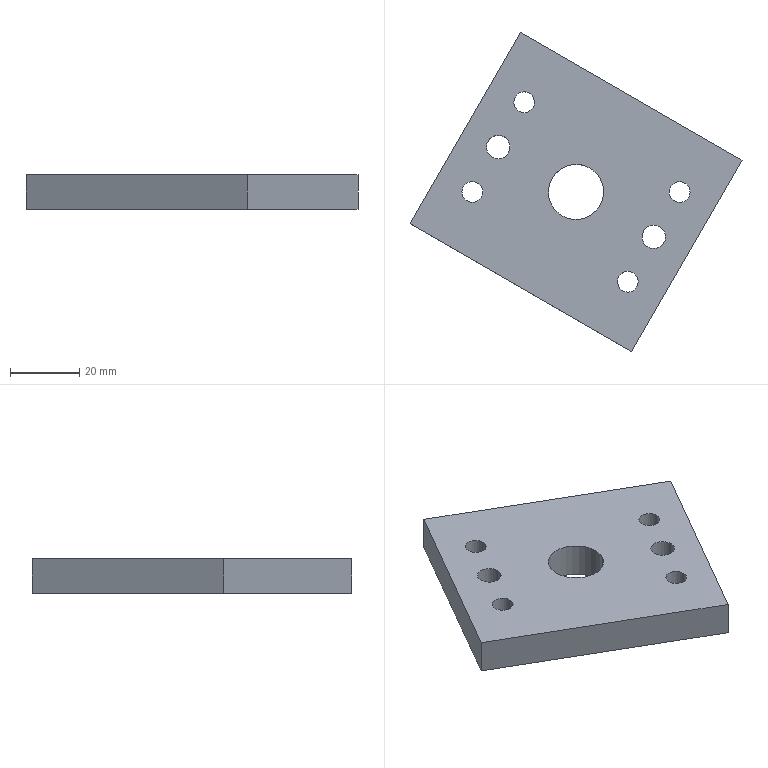Component | SolidWorks | KLHFH001LocatingPlate-1 | 1 solid | 20 faces | box 96.09 x 92.43 x 10 mm | volume 43492 mm3 | cylinder 14 | plane 6 | commonest cylinder face diameters 6 x8 6.8 x4 16 x2 | material AISI Type A2 Tool Steel
build123d program:
from build123d import *

# Parameters (mm, degrees)
SKETCH1_W                 = 74
SKETCH1_H                 = 64
BOSS_EXTRUDE1_DEPTH       = 5
SKETCH2_R                 = 8
CUT_EXTRUDE1_DEPTH        = 50.93
SIZE_MM_DOWEL_PIN_HOLE1_D = 6
CIRPATTERN1_COUNT         = 6
M8_TAPPED_HOLE2_D         = 6.8


with BuildPart() as part:
    # Sketch1 → Boss-Extrude1 (new, symmetric)
    with BuildSketch(Plane.XY):
        Rectangle(SKETCH1_W, SKETCH1_H)
    extrude(amount=BOSS_EXTRUDE1_DEPTH, both=True)

    # Sketch2 → Cut-Extrude1 (cut, through all)
    with BuildSketch(Plane.XY.offset(5)):
        Circle(SKETCH2_R)
    extrude(amount=-CUT_EXTRUDE1_DEPTH, mode=Mode.SUBTRACT)

    # Size mm Dowel Pin Hole1 (through all)
    with Locations(Plane(origin=(0, 0, -5), x_dir=(-1, 0, 0), z_dir=(0, 0, -1))):
        with Locations((-25.981, 15)):
            size_mm_dowel_pin_hole1 = Hole(SIZE_MM_DOWEL_PIN_HOLE1_D / 2)

    # CirPattern1: Size mm Dowel Pin Hole1 ×6 about axis, 2 skipped
    cirpattern1_axis = Axis((0, 0, -5), (0, 0, 1))
    add([size_mm_dowel_pin_hole1.rotate(cirpattern1_axis, i * 360 / CIRPATTERN1_COUNT) for i in range(1, CIRPATTERN1_COUNT) if i not in (1, 4)], mode=Mode.SUBTRACT)

    # M8 Tapped Hole2 (through all)
    with Locations(Plane(origin=(0, 0, -5), x_dir=(-1, 0, 0), z_dir=(0, 0, -1))):
        with Locations((25.981, 0), (-25.981, 0)):
            Hole(M8_TAPPED_HOLE2_D / 2)


solid = part.part

# Placed as in the assembly
solid = solid.moved(Location((91, 157.617, -436), (0, 0, -30)))
STEP:
#1=COLOUR_RGB('',0.7922,0.8196,0.9333);
#2=FILL_AREA_STYLE_COLOUR('',#1);
#3=FILL_AREA_STYLE('',(#2));
#4=SURFACE_STYLE_FILL_AREA(#3);
#5=SURFACE_SIDE_STYLE('',(#4));
#6=SURFACE_STYLE_USAGE(.BOTH.,#5);
#7=PRESENTATION_STYLE_ASSIGNMENT((#6));
#8=CARTESIAN_POINT('',(2.813,6.65,-16.969));
#9=VERTEX_POINT('',#8);
#10=CARTESIAN_POINT('',(2.581,6.784,-16.969));
#11=VERTEX_POINT('',#10);
#12=CARTESIAN_POINT('',(2.697,6.717,-16.969));
#13=DIRECTION('',(0.,0.,-1.));
#14=DIRECTION('',(-0.866,0.5,0.));
#15=AXIS2_PLACEMENT_3D('',#12,#13,#14);
#16=CIRCLE('',#15,0.1339);
#17=EDGE_CURVE('',#9,#11,#16,.T.);
#18=ORIENTED_EDGE('',*,*,#17,.F.);
#19=CARTESIAN_POINT('',(2.813,6.65,-17.362));
#20=VERTEX_POINT('',#19);
#21=CARTESIAN_POINT('',(2.813,6.65,-17.362));
#22=DIRECTION('',(0.,0.,-1.));
#23=VECTOR('',#22,39.37);
#24=LINE('',#21,#23);
#25=EDGE_CURVE('',#9,#20,#24,.T.);
#26=ORIENTED_EDGE('',*,*,#25,.T.);
#27=CARTESIAN_POINT('',(2.581,6.784,-17.362));
#28=VERTEX_POINT('',#27);
#29=CARTESIAN_POINT('',(2.697,6.717,-17.362));
#30=DIRECTION('',(0.,0.,-1.));
#31=DIRECTION('',(-0.866,0.5,0.));
#32=AXIS2_PLACEMENT_3D('',#29,#30,#31);
#33=CIRCLE('',#32,0.1339);
#34=EDGE_CURVE('',#20,#28,#33,.T.);
#35=ORIENTED_EDGE('',*,*,#34,.T.);
#36=CARTESIAN_POINT('',(2.581,6.784,-17.362));
#37=DIRECTION('',(0.,0.,-1.));
#38=VECTOR('',#37,39.37);
#39=LINE('',#36,#38);
#40=EDGE_CURVE('',#11,#28,#39,.T.);
#41=ORIENTED_EDGE('',*,*,#40,.F.);
#42=EDGE_LOOP('',(#18,#26,#35,#41));
#43=FACE_OUTER_BOUND('',#42,.T.);
#44=CARTESIAN_POINT('',(2.697,6.717,-17.362));
#45=DIRECTION('',(0.,0.,-1.));
#46=DIRECTION('',(-0.866,0.5,0.));
#47=AXIS2_PLACEMENT_3D('',#44,#45,#46);
#48=CYLINDRICAL_SURFACE('',#47,0.1339);
#49=ADVANCED_FACE('',(#43),#48,.F.);
#50=CARTESIAN_POINT('',(4.584,5.627,-16.969));
#51=VERTEX_POINT('',#50);
#52=CARTESIAN_POINT('',(4.353,5.761,-16.969));
#53=VERTEX_POINT('',#52);
#54=CARTESIAN_POINT('',(4.469,5.694,-16.969));
#55=DIRECTION('',(0.,0.,-1.));
#56=DIRECTION('',(-0.866,0.5,0.));
#57=AXIS2_PLACEMENT_3D('',#54,#55,#56);
#58=CIRCLE('',#57,0.1339);
#59=EDGE_CURVE('',#51,#53,#58,.T.);
#60=ORIENTED_EDGE('',*,*,#59,.F.);
#61=CARTESIAN_POINT('',(4.584,5.627,-17.362));
#62=VERTEX_POINT('',#61);
#63=CARTESIAN_POINT('',(4.584,5.627,-17.362));
#64=DIRECTION('',(0.,0.,-1.));
#65=VECTOR('',#64,39.37);
#66=LINE('',#63,#65);
#67=EDGE_CURVE('',#51,#62,#66,.T.);
#68=ORIENTED_EDGE('',*,*,#67,.T.);
#69=CARTESIAN_POINT('',(4.353,5.761,-17.362));
#70=VERTEX_POINT('',#69);
#71=CARTESIAN_POINT('',(4.469,5.694,-17.362));
#72=DIRECTION('',(0.,0.,-1.));
#73=DIRECTION('',(-0.866,0.5,0.));
#74=AXIS2_PLACEMENT_3D('',#71,#72,#73);
#75=CIRCLE('',#74,0.1339);
#76=EDGE_CURVE('',#62,#70,#75,.T.);
#77=ORIENTED_EDGE('',*,*,#76,.T.);
#78=CARTESIAN_POINT('',(4.353,5.761,-17.362));
#79=DIRECTION('',(0.,0.,-1.));
#80=VECTOR('',#79,39.37);
#81=LINE('',#78,#80);
#82=EDGE_CURVE('',#53,#70,#81,.T.);
#83=ORIENTED_EDGE('',*,*,#82,.F.);
#84=EDGE_LOOP('',(#60,#68,#77,#83));
#85=FACE_OUTER_BOUND('',#84,.T.);
#86=CARTESIAN_POINT('',(4.469,5.694,-17.362));
#87=DIRECTION('',(0.,0.,-1.));
#88=DIRECTION('',(-0.866,0.5,0.));
#89=AXIS2_PLACEMENT_3D('',#86,#87,#88);
#90=CYLINDRICAL_SURFACE('',#89,0.1339);
#91=ADVANCED_FACE('',(#85),#90,.F.);
#92=CARTESIAN_POINT('',(4.276,5.123,-16.969));
#93=VERTEX_POINT('',#92);
#94=CARTESIAN_POINT('',(4.071,5.242,-16.969));
#95=VERTEX_POINT('',#94);
#96=CARTESIAN_POINT('',(4.173,5.183,-16.969));
#97=DIRECTION('',(0.,0.,-1.));
#98=DIRECTION('',(-0.866,0.5,0.));
#99=AXIS2_PLACEMENT_3D('',#96,#97,#98);
#100=CIRCLE('',#99,0.1181);
#101=EDGE_CURVE('',#93,#95,#100,.T.);
#102=ORIENTED_EDGE('',*,*,#101,.F.);
#103=CARTESIAN_POINT('',(4.276,5.123,-17.362));
#104=VERTEX_POINT('',#103);
#105=CARTESIAN_POINT('',(4.276,5.123,-17.362));
#106=DIRECTION('',(0.,0.,-1.));
#107=VECTOR('',#106,39.37);
#108=LINE('',#105,#107);
#109=EDGE_CURVE('',#93,#104,#108,.T.);
#110=ORIENTED_EDGE('',*,*,#109,.T.);
#111=CARTESIAN_POINT('',(4.071,5.242,-17.362));
#112=VERTEX_POINT('',#111);
#113=CARTESIAN_POINT('',(4.173,5.183,-17.362));
#114=DIRECTION('',(0.,0.,-1.));
#115=DIRECTION('',(-0.866,0.5,0.));
#116=AXIS2_PLACEMENT_3D('',#113,#114,#115);
#117=CIRCLE('',#116,0.1181);
#118=EDGE_CURVE('',#104,#112,#117,.T.);
#119=ORIENTED_EDGE('',*,*,#118,.T.);
#120=CARTESIAN_POINT('',(4.071,5.242,-17.362));
#121=DIRECTION('',(0.,0.,-1.));
#122=VECTOR('',#121,39.37);
#123=LINE('',#120,#122);
#124=EDGE_CURVE('',#95,#112,#123,.T.);
#125=ORIENTED_EDGE('',*,*,#124,.F.);
#126=EDGE_LOOP('',(#102,#110,#119,#125));
#127=FACE_OUTER_BOUND('',#126,.T.);
#128=CARTESIAN_POINT('',(4.173,5.183,-17.362));
#129=DIRECTION('',(0.,0.,-1.));
#130=DIRECTION('',(-0.866,0.5,0.));
#131=AXIS2_PLACEMENT_3D('',#128,#129,#130);
#132=CYLINDRICAL_SURFACE('',#131,0.1181);
#133=ADVANCED_FACE('',(#127),#132,.F.);
#134=CARTESIAN_POINT('',(2.504,6.146,-16.969));
#135=VERTEX_POINT('',#134);
#136=CARTESIAN_POINT('',(2.299,6.264,-16.969));
#137=VERTEX_POINT('',#136);
#138=CARTESIAN_POINT('',(2.402,6.205,-16.969));
#139=DIRECTION('',(0.,0.,-1.));
#140=DIRECTION('',(-0.866,0.5,0.));
#141=AXIS2_PLACEMENT_3D('',#138,#139,#140);
#142=CIRCLE('',#141,0.1181);
#143=EDGE_CURVE('',#135,#137,#142,.T.);
#144=ORIENTED_EDGE('',*,*,#143,.F.);
#145=CARTESIAN_POINT('',(2.504,6.146,-17.362));
#146=VERTEX_POINT('',#145);
#147=CARTESIAN_POINT('',(2.504,6.146,-17.362));
#148=DIRECTION('',(0.,0.,-1.));
#149=VECTOR('',#148,39.37);
#150=LINE('',#147,#149);
#151=EDGE_CURVE('',#135,#146,#150,.T.);
#152=ORIENTED_EDGE('',*,*,#151,.T.);
#153=CARTESIAN_POINT('',(2.299,6.264,-17.362));
#154=VERTEX_POINT('',#153);
#155=CARTESIAN_POINT('',(2.402,6.205,-17.362));
#156=DIRECTION('',(0.,0.,-1.));
#157=DIRECTION('',(-0.866,0.5,0.));
#158=AXIS2_PLACEMENT_3D('',#155,#156,#157);
#159=CIRCLE('',#158,0.1181);
#160=EDGE_CURVE('',#146,#154,#159,.T.);
#161=ORIENTED_EDGE('',*,*,#160,.T.);
#162=CARTESIAN_POINT('',(2.299,6.264,-17.362));
#163=DIRECTION('',(0.,0.,-1.));
#164=VECTOR('',#163,39.37);
#165=LINE('',#162,#164);
#166=EDGE_CURVE('',#137,#154,#165,.T.);
#167=ORIENTED_EDGE('',*,*,#166,.F.);
#168=EDGE_LOOP('',(#144,#152,#161,#167));
#169=FACE_OUTER_BOUND('',#168,.T.);
#170=CARTESIAN_POINT('',(2.402,6.205,-17.362));
#171=DIRECTION('',(0.,0.,-1.));
#172=DIRECTION('',(-0.866,0.5,0.));
#173=AXIS2_PLACEMENT_3D('',#170,#171,#172);
#174=CYLINDRICAL_SURFACE('',#173,0.1181);
#175=ADVANCED_FACE('',(#169),#174,.F.);
#176=CARTESIAN_POINT('',(3.094,7.169,-16.969));
#177=VERTEX_POINT('',#176);
#178=CARTESIAN_POINT('',(2.89,7.287,-16.969));
#179=VERTEX_POINT('',#178);
#180=CARTESIAN_POINT('',(2.992,7.228,-16.969));
#181=DIRECTION('',(0.,0.,-1.));
#182=DIRECTION('',(-0.866,0.5,0.));
#183=AXIS2_PLACEMENT_3D('',#180,#181,#182);
#184=CIRCLE('',#183,0.1181);
#185=EDGE_CURVE('',#177,#179,#184,.T.);
#186=ORIENTED_EDGE('',*,*,#185,.F.);
#187=CARTESIAN_POINT('',(3.094,7.169,-17.362));
#188=VERTEX_POINT('',#187);
#189=CARTESIAN_POINT('',(3.094,7.169,-17.362));
#190=DIRECTION('',(0.,0.,-1.));
#191=VECTOR('',#190,39.37);
#192=LINE('',#189,#191);
#193=EDGE_CURVE('',#177,#188,#192,.T.);
#194=ORIENTED_EDGE('',*,*,#193,.T.);
#195=CARTESIAN_POINT('',(2.89,7.287,-17.362));
#196=VERTEX_POINT('',#195);
#197=CARTESIAN_POINT('',(2.992,7.228,-17.362));
#198=DIRECTION('',(0.,0.,-1.));
#199=DIRECTION('',(-0.866,0.5,0.));
#200=AXIS2_PLACEMENT_3D('',#197,#198,#199);
#201=CIRCLE('',#200,0.1181);
#202=EDGE_CURVE('',#188,#196,#201,.T.);
#203=ORIENTED_EDGE('',*,*,#202,.T.);
#204=CARTESIAN_POINT('',(2.89,7.287,-17.362));
#205=DIRECTION('',(0.,0.,-1.));
#206=VECTOR('',#205,39.37);
#207=LINE('',#204,#206);
#208=EDGE_CURVE('',#179,#196,#207,.T.);
#209=ORIENTED_EDGE('',*,*,#208,.F.);
#210=EDGE_LOOP('',(#186,#194,#203,#209));
#211=FACE_OUTER_BOUND('',#210,.T.);
#212=CARTESIAN_POINT('',(2.992,7.228,-17.362));
#213=DIRECTION('',(0.,0.,-1.));
#214=DIRECTION('',(-0.866,0.5,0.));
#215=AXIS2_PLACEMENT_3D('',#212,#213,#214);
#216=CYLINDRICAL_SURFACE('',#215,0.1181);
#217=ADVANCED_FACE('',(#211),#216,.F.);
#218=CARTESIAN_POINT('',(4.866,6.146,-16.969));
#219=VERTEX_POINT('',#218);
#220=CARTESIAN_POINT('',(4.661,6.264,-16.969));
#221=VERTEX_POINT('',#220);
#222=CARTESIAN_POINT('',(4.764,6.205,-16.969));
#223=DIRECTION('',(0.,0.,-1.));
#224=DIRECTION('',(-0.866,0.5,0.));
#225=AXIS2_PLACEMENT_3D('',#222,#223,#224);
#226=CIRCLE('',#225,0.1181);
#227=EDGE_CURVE('',#219,#221,#226,.T.);
#228=ORIENTED_EDGE('',*,*,#227,.F.);
#229=CARTESIAN_POINT('',(4.866,6.146,-17.362));
#230=VERTEX_POINT('',#229);
#231=CARTESIAN_POINT('',(4.866,6.146,-17.362));
#232=DIRECTION('',(0.,0.,-1.));
#233=VECTOR('',#232,39.37);
#234=LINE('',#231,#233);
#235=EDGE_CURVE('',#219,#230,#234,.T.);
#236=ORIENTED_EDGE('',*,*,#235,.T.);
#237=CARTESIAN_POINT('',(4.661,6.264,-17.362));
#238=VERTEX_POINT('',#237);
#239=CARTESIAN_POINT('',(4.764,6.205,-17.362));
#240=DIRECTION('',(0.,0.,-1.));
#241=DIRECTION('',(-0.866,0.5,0.));
#242=AXIS2_PLACEMENT_3D('',#239,#240,#241);
#243=CIRCLE('',#242,0.1181);
#244=EDGE_CURVE('',#230,#238,#243,.T.);
#245=ORIENTED_EDGE('',*,*,#244,.T.);
#246=CARTESIAN_POINT('',(4.661,6.264,-17.362));
#247=DIRECTION('',(0.,0.,-1.));
#248=VECTOR('',#247,39.37);
#249=LINE('',#246,#248);
#250=EDGE_CURVE('',#221,#238,#249,.T.);
#251=ORIENTED_EDGE('',*,*,#250,.F.);
#252=EDGE_LOOP('',(#228,#236,#245,#251));
#253=FACE_OUTER_BOUND('',#252,.T.);
#254=CARTESIAN_POINT('',(4.764,6.205,-17.362));
#255=DIRECTION('',(0.,0.,-1.));
#256=DIRECTION('',(-0.866,0.5,0.));
#257=AXIS2_PLACEMENT_3D('',#254,#255,#256);
#258=CYLINDRICAL_SURFACE('',#257,0.1181);
#259=ADVANCED_FACE('',(#253),#258,.F.);
#260=CARTESIAN_POINT('',(3.31,6.363,-17.362));
#261=VERTEX_POINT('',#260);
#262=CARTESIAN_POINT('',(3.855,6.048,-17.362));
#263=VERTEX_POINT('',#262);
#264=CARTESIAN_POINT('',(3.583,6.205,-17.362));
#265=DIRECTION('',(0.,0.,1.));
#266=DIRECTION('',(0.866,-0.5,0.));
#267=AXIS2_PLACEMENT_3D('',#264,#265,#266);
#268=CIRCLE('',#267,0.315);
#269=EDGE_CURVE('',#261,#263,#268,.T.);
#270=ORIENTED_EDGE('',*,*,#269,.F.);
#271=CARTESIAN_POINT('',(3.31,6.363,-16.969));
#272=VERTEX_POINT('',#271);
#273=CARTESIAN_POINT('',(3.31,6.363,-17.362));
#274=DIRECTION('',(0.,0.,1.));
#275=VECTOR('',#274,39.37);
#276=LINE('',#273,#275);
#277=EDGE_CURVE('',#261,#272,#276,.T.);
#278=ORIENTED_EDGE('',*,*,#277,.T.);
#279=CARTESIAN_POINT('',(3.855,6.048,-16.969));
#280=VERTEX_POINT('',#279);
#281=CARTESIAN_POINT('',(3.583,6.205,-16.969));
#282=DIRECTION('',(0.,0.,1.));
#283=DIRECTION('',(0.866,-0.5,0.));
#284=AXIS2_PLACEMENT_3D('',#281,#282,#283);
#285=CIRCLE('',#284,0.315);
#286=EDGE_CURVE('',#272,#280,#285,.T.);
#287=ORIENTED_EDGE('',*,*,#286,.T.);
#288=CARTESIAN_POINT('',(3.855,6.048,-17.362));
#289=DIRECTION('',(0.,0.,1.));
#290=VECTOR('',#289,39.37);
#291=LINE('',#288,#290);
#292=EDGE_CURVE('',#263,#280,#291,.T.);
#293=ORIENTED_EDGE('',*,*,#292,.F.);
#294=EDGE_LOOP('',(#270,#278,#287,#293));
#295=FACE_OUTER_BOUND('',#294,.T.);
#296=CARTESIAN_POINT('',(3.583,6.205,-17.362));
#297=DIRECTION('',(0.,0.,1.));
#298=DIRECTION('',(0.866,-0.5,0.));
#299=AXIS2_PLACEMENT_3D('',#296,#297,#298);
#300=CYLINDRICAL_SURFACE('',#299,0.315);
#301=ADVANCED_FACE('',(#295),#300,.F.);
#302=CARTESIAN_POINT('',(2.951,8.025,-17.362));
#303=VERTEX_POINT('',#302);
#304=CARTESIAN_POINT('',(1.691,5.843,-17.362));
#305=VERTEX_POINT('',#304);
#306=CARTESIAN_POINT('',(2.951,8.025,-17.362));
#307=DIRECTION('',(-0.5,-0.866,0.));
#308=VECTOR('',#307,39.37);
#309=LINE('',#306,#308);
#310=EDGE_CURVE('',#303,#305,#309,.T.);
#311=ORIENTED_EDGE('',*,*,#310,.T.);
#312=CARTESIAN_POINT('',(1.691,5.843,-16.969));
#313=VERTEX_POINT('',#312);
#314=CARTESIAN_POINT('',(1.691,5.843,-16.969));
#315=DIRECTION('',(0.,0.,-1.));
#316=VECTOR('',#315,39.37);
#317=LINE('',#314,#316);
#318=EDGE_CURVE('',#313,#305,#317,.T.);
#319=ORIENTED_EDGE('',*,*,#318,.F.);
#320=CARTESIAN_POINT('',(2.951,8.025,-16.969));
#321=VERTEX_POINT('',#320);
#322=CARTESIAN_POINT('',(2.951,8.025,-16.969));
#323=DIRECTION('',(-0.5,-0.866,0.));
#324=VECTOR('',#323,39.37);
#325=LINE('',#322,#324);
#326=EDGE_CURVE('',#321,#313,#325,.T.);
#327=ORIENTED_EDGE('',*,*,#326,.F.);
#328=CARTESIAN_POINT('',(2.951,8.025,-16.969));
#329=DIRECTION('',(0.,0.,-1.));
#330=VECTOR('',#329,39.37);
#331=LINE('',#328,#330);
#332=EDGE_CURVE('',#321,#303,#331,.T.);
#333=ORIENTED_EDGE('',*,*,#332,.T.);
#334=EDGE_LOOP('',(#311,#319,#327,#333));
#335=FACE_OUTER_BOUND('',#334,.T.);
#336=CARTESIAN_POINT('',(2.951,8.025,-16.969));
#337=DIRECTION('',(0.866,-0.5,0.));
#338=DIRECTION('',(0.5,0.866,0.));
#339=AXIS2_PLACEMENT_3D('',#336,#337,#338);
#340=PLANE('',#339);
#341=ADVANCED_FACE('',(#335),#340,.F.);
#342=CARTESIAN_POINT('',(4.214,4.386,-17.362));
#343=VERTEX_POINT('',#342);
#344=CARTESIAN_POINT('',(4.214,4.386,-17.362));
#345=DIRECTION('',(0.866,-0.5,0.));
#346=VECTOR('',#345,39.37);
#347=LINE('',#344,#346);
#348=EDGE_CURVE('',#305,#343,#347,.T.);
#349=ORIENTED_EDGE('',*,*,#348,.T.);
#350=CARTESIAN_POINT('',(4.214,4.386,-16.969));
#351=VERTEX_POINT('',#350);
#352=CARTESIAN_POINT('',(4.214,4.386,-16.969));
#353=DIRECTION('',(0.,0.,-1.));
#354=VECTOR('',#353,39.37);
#355=LINE('',#352,#354);
#356=EDGE_CURVE('',#351,#343,#355,.T.);
#357=ORIENTED_EDGE('',*,*,#356,.F.);
#358=CARTESIAN_POINT('',(4.214,4.386,-16.969));
#359=DIRECTION('',(0.866,-0.5,0.));
#360=VECTOR('',#359,39.37);
#361=LINE('',#358,#360);
#362=EDGE_CURVE('',#313,#351,#361,.T.);
#363=ORIENTED_EDGE('',*,*,#362,.F.);
#364=ORIENTED_EDGE('',*,*,#318,.T.);
#365=EDGE_LOOP('',(#349,#357,#363,#364));
#366=FACE_OUTER_BOUND('',#365,.T.);
#367=CARTESIAN_POINT('',(4.214,4.386,-16.969));
#368=DIRECTION('',(0.5,0.866,0.));
#369=DIRECTION('',(-0.866,0.5,0.));
#370=AXIS2_PLACEMENT_3D('',#367,#368,#369);
#371=PLANE('',#370);
#372=ADVANCED_FACE('',(#366),#371,.F.);
#373=CARTESIAN_POINT('',(5.474,6.568,-17.362));
#374=VERTEX_POINT('',#373);
#375=CARTESIAN_POINT('',(5.474,6.568,-17.362));
#376=DIRECTION('',(0.5,0.866,0.));
#377=VECTOR('',#376,39.37);
#378=LINE('',#375,#377);
#379=EDGE_CURVE('',#343,#374,#378,.T.);
#380=ORIENTED_EDGE('',*,*,#379,.T.);
#381=CARTESIAN_POINT('',(5.474,6.568,-16.969));
#382=VERTEX_POINT('',#381);
#383=CARTESIAN_POINT('',(5.474,6.568,-16.969));
#384=DIRECTION('',(0.,0.,-1.));
#385=VECTOR('',#384,39.37);
#386=LINE('',#383,#385);
#387=EDGE_CURVE('',#382,#374,#386,.T.);
#388=ORIENTED_EDGE('',*,*,#387,.F.);
#389=CARTESIAN_POINT('',(5.474,6.568,-16.969));
#390=DIRECTION('',(0.5,0.866,0.));
#391=VECTOR('',#390,39.37);
#392=LINE('',#389,#391);
#393=EDGE_CURVE('',#351,#382,#392,.T.);
#394=ORIENTED_EDGE('',*,*,#393,.F.);
#395=ORIENTED_EDGE('',*,*,#356,.T.);
#396=EDGE_LOOP('',(#380,#388,#394,#395));
#397=FACE_OUTER_BOUND('',#396,.T.);
#398=CARTESIAN_POINT('',(5.474,6.568,-16.969));
#399=DIRECTION('',(-0.866,0.5,0.));
#400=DIRECTION('',(-0.5,-0.866,0.));
#401=AXIS2_PLACEMENT_3D('',#398,#399,#400);
#402=PLANE('',#401);
#403=ADVANCED_FACE('',(#397),#402,.F.);
#404=CARTESIAN_POINT('',(5.474,6.568,-17.362));
#405=DIRECTION('',(-0.866,0.5,0.));
#406=VECTOR('',#405,39.37);
#407=LINE('',#404,#406);
#408=EDGE_CURVE('',#374,#303,#407,.T.);
#409=ORIENTED_EDGE('',*,*,#408,.T.);
#410=ORIENTED_EDGE('',*,*,#332,.F.);
#411=CARTESIAN_POINT('',(5.474,6.568,-16.969));
#412=DIRECTION('',(-0.866,0.5,0.));
#413=VECTOR('',#412,39.37);
#414=LINE('',#411,#413);
#415=EDGE_CURVE('',#382,#321,#414,.T.);
#416=ORIENTED_EDGE('',*,*,#415,.F.);
#417=ORIENTED_EDGE('',*,*,#387,.T.);
#418=EDGE_LOOP('',(#409,#410,#416,#417));
#419=FACE_OUTER_BOUND('',#418,.T.);
#420=CARTESIAN_POINT('',(5.474,6.568,-16.969));
#421=DIRECTION('',(-0.5,-0.866,0.));
#422=DIRECTION('',(0.866,-0.5,0.));
#423=AXIS2_PLACEMENT_3D('',#420,#421,#422);
#424=PLANE('',#423);
#425=ADVANCED_FACE('',(#419),#424,.F.);
#426=CARTESIAN_POINT('',(2.697,6.717,-16.969));
#427=DIRECTION('',(0.,0.,-1.));
#428=DIRECTION('',(-0.866,0.5,0.));
#429=AXIS2_PLACEMENT_3D('',#426,#427,#428);
#430=CIRCLE('',#429,0.1339);
#431=EDGE_CURVE('',#11,#9,#430,.T.);
#432=ORIENTED_EDGE('',*,*,#431,.T.);
#433=ORIENTED_EDGE('',*,*,#17,.T.);
#434=EDGE_LOOP('',(#432,#433));
#435=FACE_BOUND('',#434,.T.);
#436=CARTESIAN_POINT('',(4.469,5.694,-16.969));
#437=DIRECTION('',(0.,0.,-1.));
#438=DIRECTION('',(-0.866,0.5,0.));
#439=AXIS2_PLACEMENT_3D('',#436,#437,#438);
#440=CIRCLE('',#439,0.1339);
#441=EDGE_CURVE('',#53,#51,#440,.T.);
#442=ORIENTED_EDGE('',*,*,#441,.T.);
#443=ORIENTED_EDGE('',*,*,#59,.T.);
#444=EDGE_LOOP('',(#442,#443));
#445=FACE_BOUND('',#444,.T.);
#446=CARTESIAN_POINT('',(4.173,5.183,-16.969));
#447=DIRECTION('',(0.,0.,-1.));
#448=DIRECTION('',(-0.866,0.5,0.));
#449=AXIS2_PLACEMENT_3D('',#446,#447,#448);
#450=CIRCLE('',#449,0.1181);
#451=EDGE_CURVE('',#95,#93,#450,.T.);
#452=ORIENTED_EDGE('',*,*,#451,.T.);
#453=ORIENTED_EDGE('',*,*,#101,.T.);
#454=EDGE_LOOP('',(#452,#453));
#455=FACE_BOUND('',#454,.T.);
#456=CARTESIAN_POINT('',(2.402,6.205,-16.969));
#457=DIRECTION('',(0.,0.,-1.));
#458=DIRECTION('',(-0.866,0.5,0.));
#459=AXIS2_PLACEMENT_3D('',#456,#457,#458);
#460=CIRCLE('',#459,0.1181);
#461=EDGE_CURVE('',#137,#135,#460,.T.);
#462=ORIENTED_EDGE('',*,*,#461,.T.);
#463=ORIENTED_EDGE('',*,*,#143,.T.);
#464=EDGE_LOOP('',(#462,#463));
#465=FACE_BOUND('',#464,.T.);
#466=CARTESIAN_POINT('',(2.992,7.228,-16.969));
#467=DIRECTION('',(0.,0.,-1.));
#468=DIRECTION('',(-0.866,0.5,0.));
#469=AXIS2_PLACEMENT_3D('',#466,#467,#468);
#470=CIRCLE('',#469,0.1181);
#471=EDGE_CURVE('',#179,#177,#470,.T.);
#472=ORIENTED_EDGE('',*,*,#471,.T.);
#473=ORIENTED_EDGE('',*,*,#185,.T.);
#474=EDGE_LOOP('',(#472,#473));
#475=FACE_BOUND('',#474,.T.);
#476=CARTESIAN_POINT('',(4.764,6.205,-16.969));
#477=DIRECTION('',(0.,0.,-1.));
#478=DIRECTION('',(-0.866,0.5,0.));
#479=AXIS2_PLACEMENT_3D('',#476,#477,#478);
#480=CIRCLE('',#479,0.1181);
#481=EDGE_CURVE('',#221,#219,#480,.T.);
#482=ORIENTED_EDGE('',*,*,#481,.T.);
#483=ORIENTED_EDGE('',*,*,#227,.T.);
#484=EDGE_LOOP('',(#482,#483));
#485=FACE_BOUND('',#484,.T.);
#486=CARTESIAN_POINT('',(3.583,6.205,-16.969));
#487=DIRECTION('',(0.,0.,1.));
#488=DIRECTION('',(0.866,-0.5,0.));
#489=AXIS2_PLACEMENT_3D('',#486,#487,#488);
#490=CIRCLE('',#489,0.315);
#491=EDGE_CURVE('',#280,#272,#490,.T.);
#492=ORIENTED_EDGE('',*,*,#491,.F.);
#493=ORIENTED_EDGE('',*,*,#286,.F.);
#494=EDGE_LOOP('',(#492,#493));
#495=FACE_BOUND('',#494,.T.);
#496=ORIENTED_EDGE('',*,*,#326,.T.);
#497=ORIENTED_EDGE('',*,*,#362,.T.);
#498=ORIENTED_EDGE('',*,*,#393,.T.);
#499=ORIENTED_EDGE('',*,*,#415,.T.);
#500=EDGE_LOOP('',(#496,#497,#498,#499));
#501=FACE_OUTER_BOUND('',#500,.T.);
#502=CARTESIAN_POINT('',(3.583,6.205,-16.969));
#503=DIRECTION('',(0.,0.,-1.));
#504=DIRECTION('',(-0.866,0.5,0.));
#505=AXIS2_PLACEMENT_3D('',#502,#503,#504);
#506=PLANE('',#505);
#507=ADVANCED_FACE('',(#435,#445,#455,#465,#475,#485,#495,#501),#506,.F.);
#508=CARTESIAN_POINT('',(2.697,6.717,-17.362));
#509=DIRECTION('',(0.,0.,-1.));
#510=DIRECTION('',(-0.866,0.5,0.));
#511=AXIS2_PLACEMENT_3D('',#508,#509,#510);
#512=CIRCLE('',#511,0.1339);
#513=EDGE_CURVE('',#28,#20,#512,.T.);
#514=ORIENTED_EDGE('',*,*,#513,.F.);
#515=ORIENTED_EDGE('',*,*,#34,.F.);
#516=EDGE_LOOP('',(#514,#515));
#517=FACE_BOUND('',#516,.T.);
#518=CARTESIAN_POINT('',(4.469,5.694,-17.362));
#519=DIRECTION('',(0.,0.,-1.));
#520=DIRECTION('',(-0.866,0.5,0.));
#521=AXIS2_PLACEMENT_3D('',#518,#519,#520);
#522=CIRCLE('',#521,0.1339);
#523=EDGE_CURVE('',#70,#62,#522,.T.);
#524=ORIENTED_EDGE('',*,*,#523,.F.);
#525=ORIENTED_EDGE('',*,*,#76,.F.);
#526=EDGE_LOOP('',(#524,#525));
#527=FACE_BOUND('',#526,.T.);
#528=CARTESIAN_POINT('',(4.173,5.183,-17.362));
#529=DIRECTION('',(0.,0.,-1.));
#530=DIRECTION('',(-0.866,0.5,0.));
#531=AXIS2_PLACEMENT_3D('',#528,#529,#530);
#532=CIRCLE('',#531,0.1181);
#533=EDGE_CURVE('',#112,#104,#532,.T.);
#534=ORIENTED_EDGE('',*,*,#533,.F.);
#535=ORIENTED_EDGE('',*,*,#118,.F.);
#536=EDGE_LOOP('',(#534,#535));
#537=FACE_BOUND('',#536,.T.);
#538=CARTESIAN_POINT('',(2.402,6.205,-17.362));
#539=DIRECTION('',(0.,0.,-1.));
#540=DIRECTION('',(-0.866,0.5,0.));
#541=AXIS2_PLACEMENT_3D('',#538,#539,#540);
#542=CIRCLE('',#541,0.1181);
#543=EDGE_CURVE('',#154,#146,#542,.T.);
#544=ORIENTED_EDGE('',*,*,#543,.F.);
#545=ORIENTED_EDGE('',*,*,#160,.F.);
#546=EDGE_LOOP('',(#544,#545));
#547=FACE_BOUND('',#546,.T.);
#548=CARTESIAN_POINT('',(2.992,7.228,-17.362));
#549=DIRECTION('',(0.,0.,-1.));
#550=DIRECTION('',(-0.866,0.5,0.));
#551=AXIS2_PLACEMENT_3D('',#548,#549,#550);
#552=CIRCLE('',#551,0.1181);
#553=EDGE_CURVE('',#196,#188,#552,.T.);
#554=ORIENTED_EDGE('',*,*,#553,.F.);
#555=ORIENTED_EDGE('',*,*,#202,.F.);
#556=EDGE_LOOP('',(#554,#555));
#557=FACE_BOUND('',#556,.T.);
#558=CARTESIAN_POINT('',(4.764,6.205,-17.362));
#559=DIRECTION('',(0.,0.,-1.));
#560=DIRECTION('',(-0.866,0.5,0.));
#561=AXIS2_PLACEMENT_3D('',#558,#559,#560);
#562=CIRCLE('',#561,0.1181);
#563=EDGE_CURVE('',#238,#230,#562,.T.);
#564=ORIENTED_EDGE('',*,*,#563,.F.);
#565=ORIENTED_EDGE('',*,*,#244,.F.);
#566=EDGE_LOOP('',(#564,#565));
#567=FACE_BOUND('',#566,.T.);
#568=CARTESIAN_POINT('',(3.583,6.205,-17.362));
#569=DIRECTION('',(0.,0.,1.));
#570=DIRECTION('',(0.866,-0.5,0.));
#571=AXIS2_PLACEMENT_3D('',#568,#569,#570);
#572=CIRCLE('',#571,0.315);
#573=EDGE_CURVE('',#263,#261,#572,.T.);
#574=ORIENTED_EDGE('',*,*,#573,.T.);
#575=ORIENTED_EDGE('',*,*,#269,.T.);
#576=EDGE_LOOP('',(#574,#575));
#577=FACE_BOUND('',#576,.T.);
#578=ORIENTED_EDGE('',*,*,#310,.F.);
#579=ORIENTED_EDGE('',*,*,#408,.F.);
#580=ORIENTED_EDGE('',*,*,#379,.F.);
#581=ORIENTED_EDGE('',*,*,#348,.F.);
#582=EDGE_LOOP('',(#578,#579,#580,#581));
#583=FACE_OUTER_BOUND('',#582,.T.);
#584=CARTESIAN_POINT('',(3.583,6.205,-17.362));
#585=DIRECTION('',(0.,0.,-1.));
#586=DIRECTION('',(-0.866,0.5,0.));
#587=AXIS2_PLACEMENT_3D('',#584,#585,#586);
#588=PLANE('',#587);
#589=ADVANCED_FACE('',(#517,#527,#537,#547,#557,#567,#577,#583),#588,.T.);
#590=ORIENTED_EDGE('',*,*,#277,.F.);
#591=ORIENTED_EDGE('',*,*,#573,.F.);
#592=ORIENTED_EDGE('',*,*,#292,.T.);
#593=ORIENTED_EDGE('',*,*,#491,.T.);
#594=EDGE_LOOP('',(#590,#591,#592,#593));
#595=FACE_OUTER_BOUND('',#594,.T.);
#596=CARTESIAN_POINT('',(3.583,6.205,-17.362));
#597=DIRECTION('',(0.,0.,1.));
#598=DIRECTION('',(0.866,-0.5,0.));
#599=AXIS2_PLACEMENT_3D('',#596,#597,#598);
#600=CYLINDRICAL_SURFACE('',#599,0.315);
#601=ADVANCED_FACE('',(#595),#600,.F.);
#602=ORIENTED_EDGE('',*,*,#235,.F.);
#603=ORIENTED_EDGE('',*,*,#481,.F.);
#604=ORIENTED_EDGE('',*,*,#250,.T.);
#605=ORIENTED_EDGE('',*,*,#563,.T.);
#606=EDGE_LOOP('',(#602,#603,#604,#605));
#607=FACE_OUTER_BOUND('',#606,.T.);
#608=CARTESIAN_POINT('',(4.764,6.205,-17.362));
#609=DIRECTION('',(0.,0.,-1.));
#610=DIRECTION('',(-0.866,0.5,0.));
#611=AXIS2_PLACEMENT_3D('',#608,#609,#610);
#612=CYLINDRICAL_SURFACE('',#611,0.1181);
#613=ADVANCED_FACE('',(#607),#612,.F.);
#614=ORIENTED_EDGE('',*,*,#193,.F.);
#615=ORIENTED_EDGE('',*,*,#471,.F.);
#616=ORIENTED_EDGE('',*,*,#208,.T.);
#617=ORIENTED_EDGE('',*,*,#553,.T.);
#618=EDGE_LOOP('',(#614,#615,#616,#617));
#619=FACE_OUTER_BOUND('',#618,.T.);
#620=CARTESIAN_POINT('',(2.992,7.228,-17.362));
#621=DIRECTION('',(0.,0.,-1.));
#622=DIRECTION('',(-0.866,0.5,0.));
#623=AXIS2_PLACEMENT_3D('',#620,#621,#622);
#624=CYLINDRICAL_SURFACE('',#623,0.1181);
#625=ADVANCED_FACE('',(#619),#624,.F.);
#626=ORIENTED_EDGE('',*,*,#151,.F.);
#627=ORIENTED_EDGE('',*,*,#461,.F.);
#628=ORIENTED_EDGE('',*,*,#166,.T.);
#629=ORIENTED_EDGE('',*,*,#543,.T.);
#630=EDGE_LOOP('',(#626,#627,#628,#629));
#631=FACE_OUTER_BOUND('',#630,.T.);
#632=CARTESIAN_POINT('',(2.402,6.205,-17.362));
#633=DIRECTION('',(0.,0.,-1.));
#634=DIRECTION('',(-0.866,0.5,0.));
#635=AXIS2_PLACEMENT_3D('',#632,#633,#634);
#636=CYLINDRICAL_SURFACE('',#635,0.1181);
#637=ADVANCED_FACE('',(#631),#636,.F.);
#638=ORIENTED_EDGE('',*,*,#109,.F.);
#639=ORIENTED_EDGE('',*,*,#451,.F.);
#640=ORIENTED_EDGE('',*,*,#124,.T.);
#641=ORIENTED_EDGE('',*,*,#533,.T.);
#642=EDGE_LOOP('',(#638,#639,#640,#641));
#643=FACE_OUTER_BOUND('',#642,.T.);
#644=CARTESIAN_POINT('',(4.173,5.183,-17.362));
#645=DIRECTION('',(0.,0.,-1.));
#646=DIRECTION('',(-0.866,0.5,0.));
#647=AXIS2_PLACEMENT_3D('',#644,#645,#646);
#648=CYLINDRICAL_SURFACE('',#647,0.1181);
#649=ADVANCED_FACE('',(#643),#648,.F.);
#650=ORIENTED_EDGE('',*,*,#67,.F.);
#651=ORIENTED_EDGE('',*,*,#441,.F.);
#652=ORIENTED_EDGE('',*,*,#82,.T.);
#653=ORIENTED_EDGE('',*,*,#523,.T.);
#654=EDGE_LOOP('',(#650,#651,#652,#653));
#655=FACE_OUTER_BOUND('',#654,.T.);
#656=CARTESIAN_POINT('',(4.469,5.694,-17.362));
#657=DIRECTION('',(0.,0.,-1.));
#658=DIRECTION('',(-0.866,0.5,0.));
#659=AXIS2_PLACEMENT_3D('',#656,#657,#658);
#660=CYLINDRICAL_SURFACE('',#659,0.1339);
#661=ADVANCED_FACE('',(#655),#660,.F.);
#662=ORIENTED_EDGE('',*,*,#25,.F.);
#663=ORIENTED_EDGE('',*,*,#431,.F.);
#664=ORIENTED_EDGE('',*,*,#40,.T.);
#665=ORIENTED_EDGE('',*,*,#513,.T.);
#666=EDGE_LOOP('',(#662,#663,#664,#665));
#667=FACE_OUTER_BOUND('',#666,.T.);
#668=CARTESIAN_POINT('',(2.697,6.717,-17.362));
#669=DIRECTION('',(0.,0.,-1.));
#670=DIRECTION('',(-0.866,0.5,0.));
#671=AXIS2_PLACEMENT_3D('',#668,#669,#670);
#672=CYLINDRICAL_SURFACE('',#671,0.1339);
#673=ADVANCED_FACE('',(#667),#672,.F.);
#674=CLOSED_SHELL('',(#49,#91,#133,#175,#217,#259,#301,#341,#372,#403,#425,#507,#589,#601,#613,#625,#637,#649,#661,#673));
#675=MANIFOLD_SOLID_BREP('',#674);
#676=STYLED_ITEM('',(#7),#675);
#677=(LENGTH_UNIT()NAMED_UNIT(*)SI_UNIT($,.METRE.));
#678=LENGTH_MEASURE_WITH_UNIT(LENGTH_MEASURE(0.0254),#677);
#679=DIMENSIONAL_EXPONENTS(1.,0.,0.,0.,0.,0.,0.);
#680=(CONVERSION_BASED_UNIT('',#678)LENGTH_UNIT()NAMED_UNIT(#679));
#681=UNCERTAINTY_MEASURE_WITH_UNIT(LENGTH_MEASURE(0.00001),#680,'','');
#682=(NAMED_UNIT(*)PLANE_ANGLE_UNIT()SI_UNIT($,.RADIAN.));
#683=(NAMED_UNIT(*)SI_UNIT($,.STERADIAN.)SOLID_ANGLE_UNIT());
#684=(GEOMETRIC_REPRESENTATION_CONTEXT(3)GLOBAL_UNCERTAINTY_ASSIGNED_CONTEXT((#681))GLOBAL_UNIT_ASSIGNED_CONTEXT((#680,#682,#683))REPRESENTATION_CONTEXT('',''));
#685=MECHANICAL_DESIGN_GEOMETRIC_PRESENTATION_REPRESENTATION('',(#676),#684);
#686=PRESENTATION_LAYER_ASSIGNMENT('','',(#676));
#687=CARTESIAN_POINT('',(0.,0.,0.));
#688=DIRECTION('',(0.,0.,1.));
#689=DIRECTION('',(1.,0.,0.));
#690=AXIS2_PLACEMENT_3D('',#687,#688,#689);
#691=(LENGTH_UNIT()NAMED_UNIT(*)SI_UNIT($,.METRE.));
#692=LENGTH_MEASURE_WITH_UNIT(LENGTH_MEASURE(0.0254),#691);
#693=DIMENSIONAL_EXPONENTS(1.,0.,0.,0.,0.,0.,0.);
#694=(CONVERSION_BASED_UNIT('',#692)LENGTH_UNIT()NAMED_UNIT(#693));
#695=UNCERTAINTY_MEASURE_WITH_UNIT(LENGTH_MEASURE(0.00001),#694,'','');
#696=(NAMED_UNIT(*)PLANE_ANGLE_UNIT()SI_UNIT($,.RADIAN.));
#697=(NAMED_UNIT(*)SI_UNIT($,.STERADIAN.)SOLID_ANGLE_UNIT());
#698=(GEOMETRIC_REPRESENTATION_CONTEXT(3)GLOBAL_UNCERTAINTY_ASSIGNED_CONTEXT((#695))GLOBAL_UNIT_ASSIGNED_CONTEXT((#694,#696,#697))REPRESENTATION_CONTEXT('',''));
#699=ADVANCED_BREP_SHAPE_REPRESENTATION('',(#675,#690),#698);